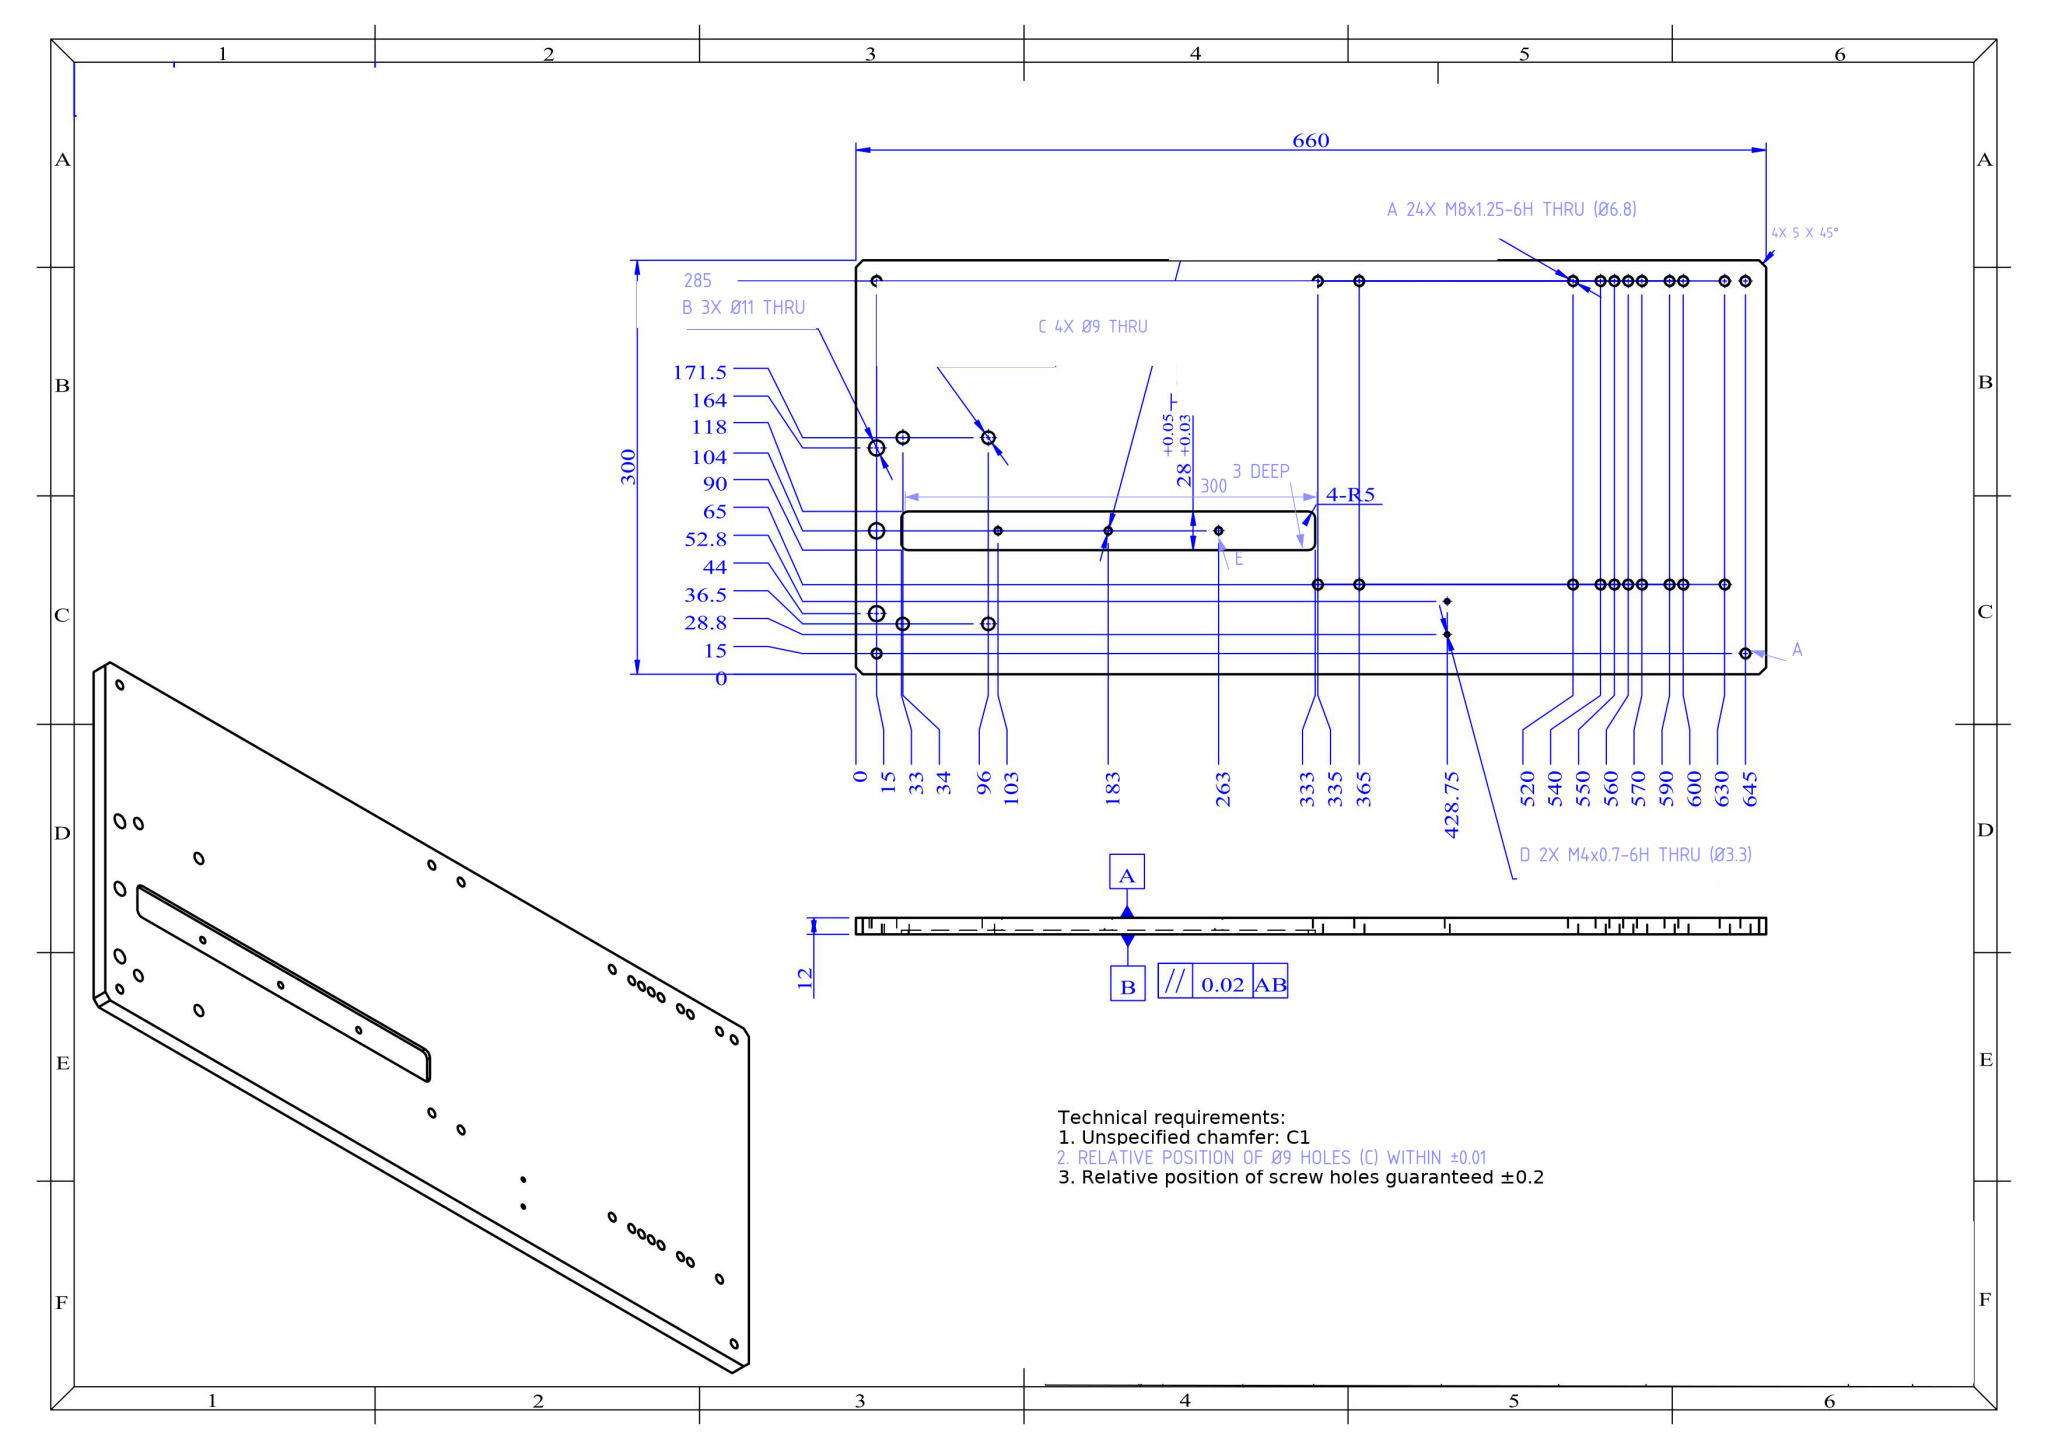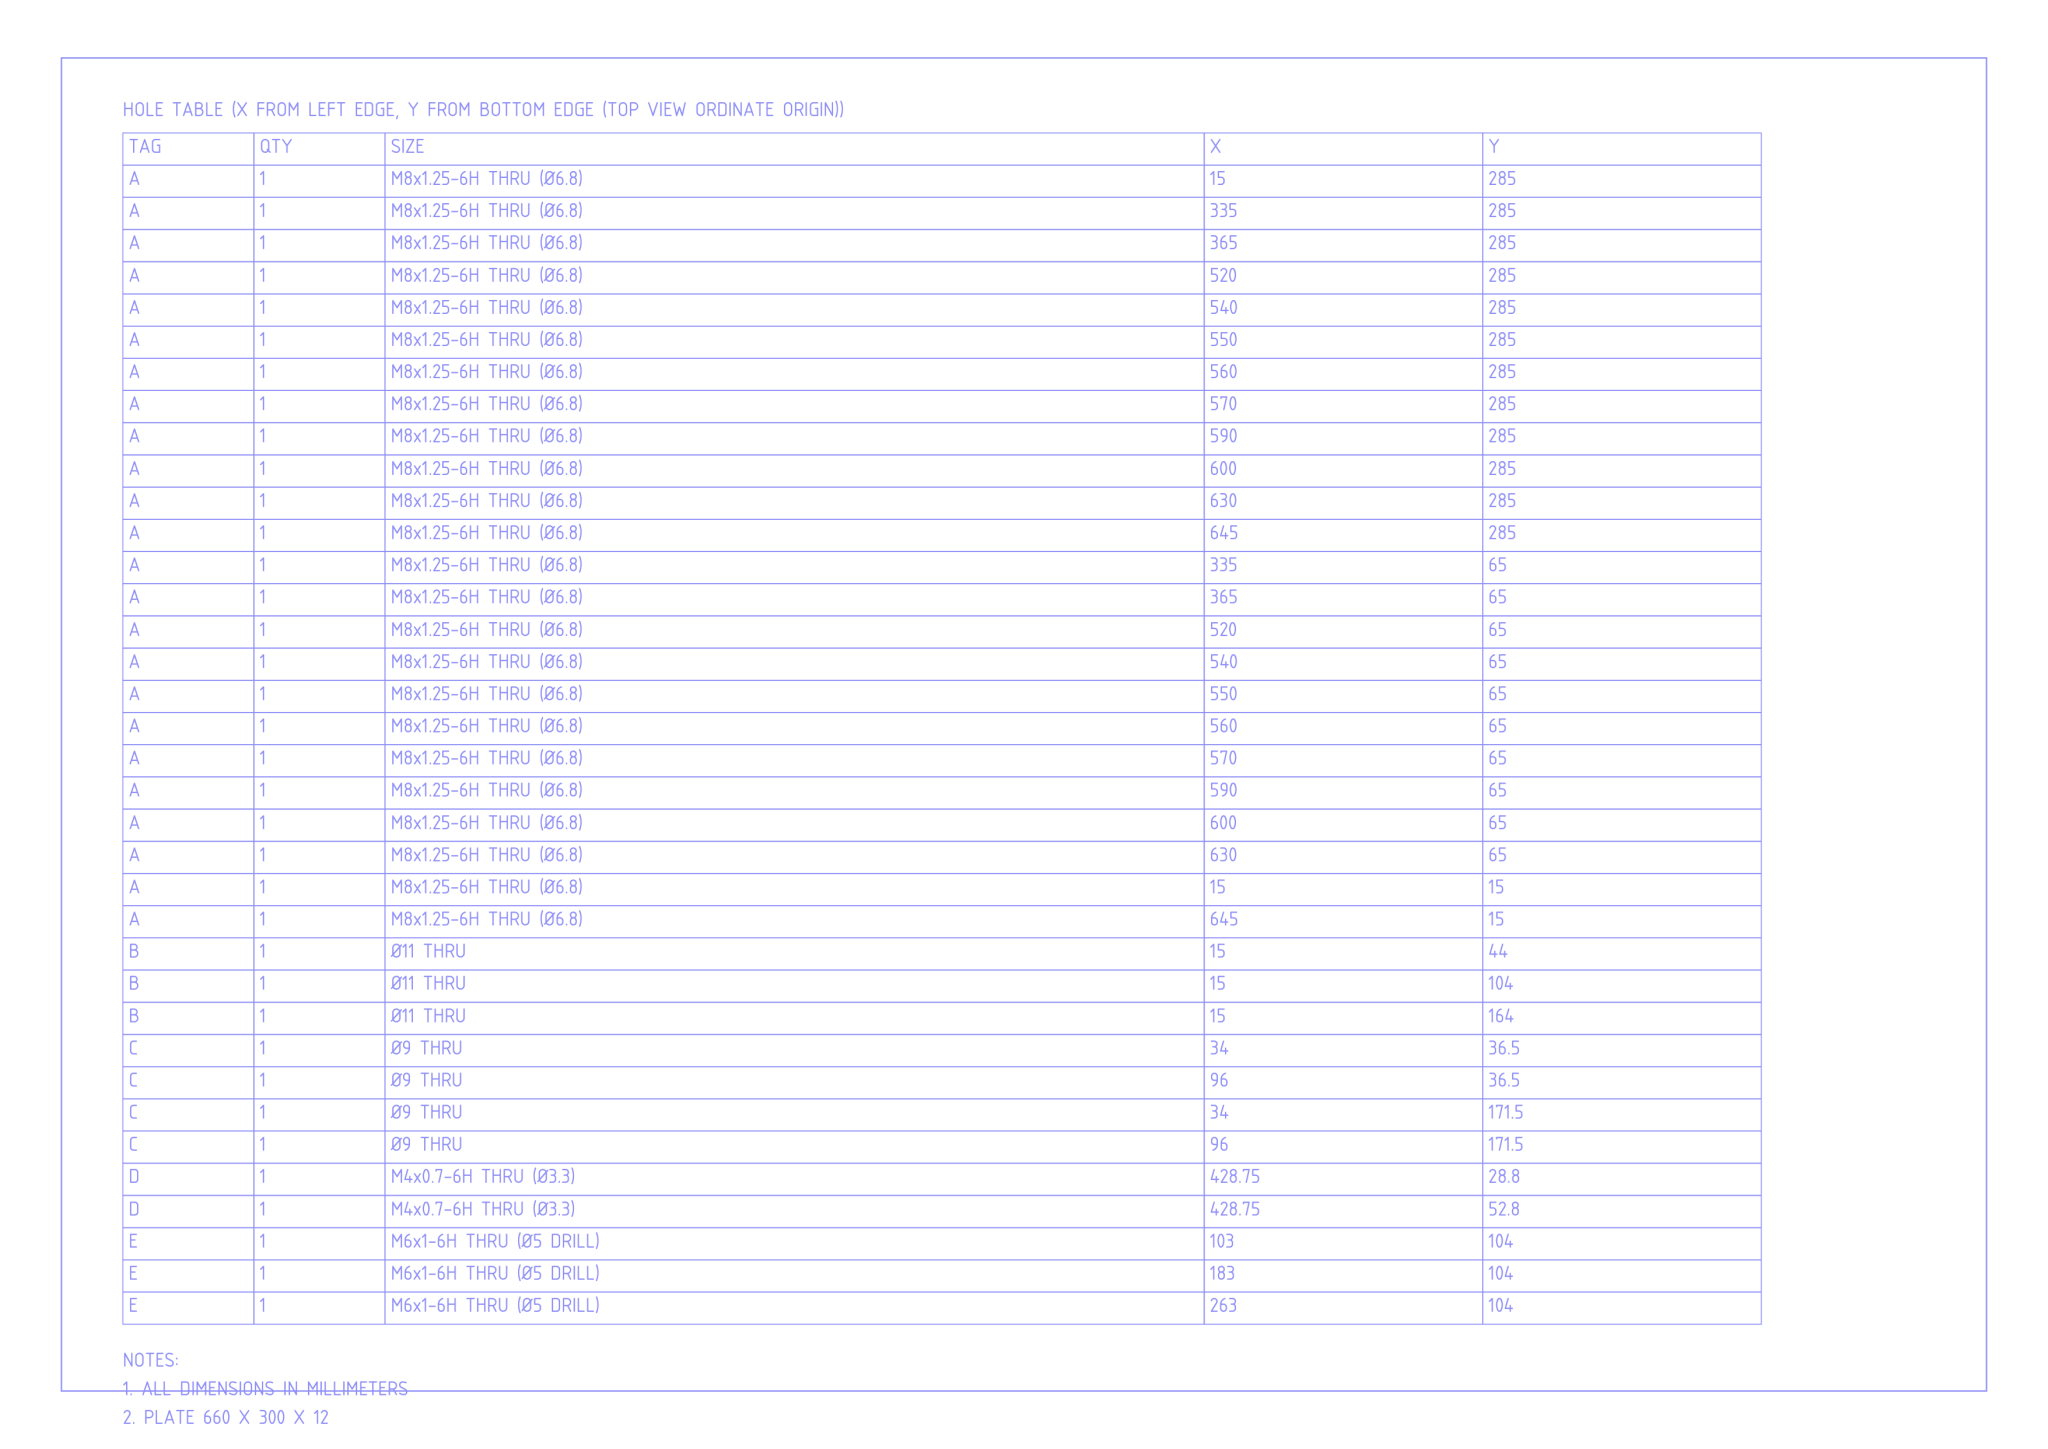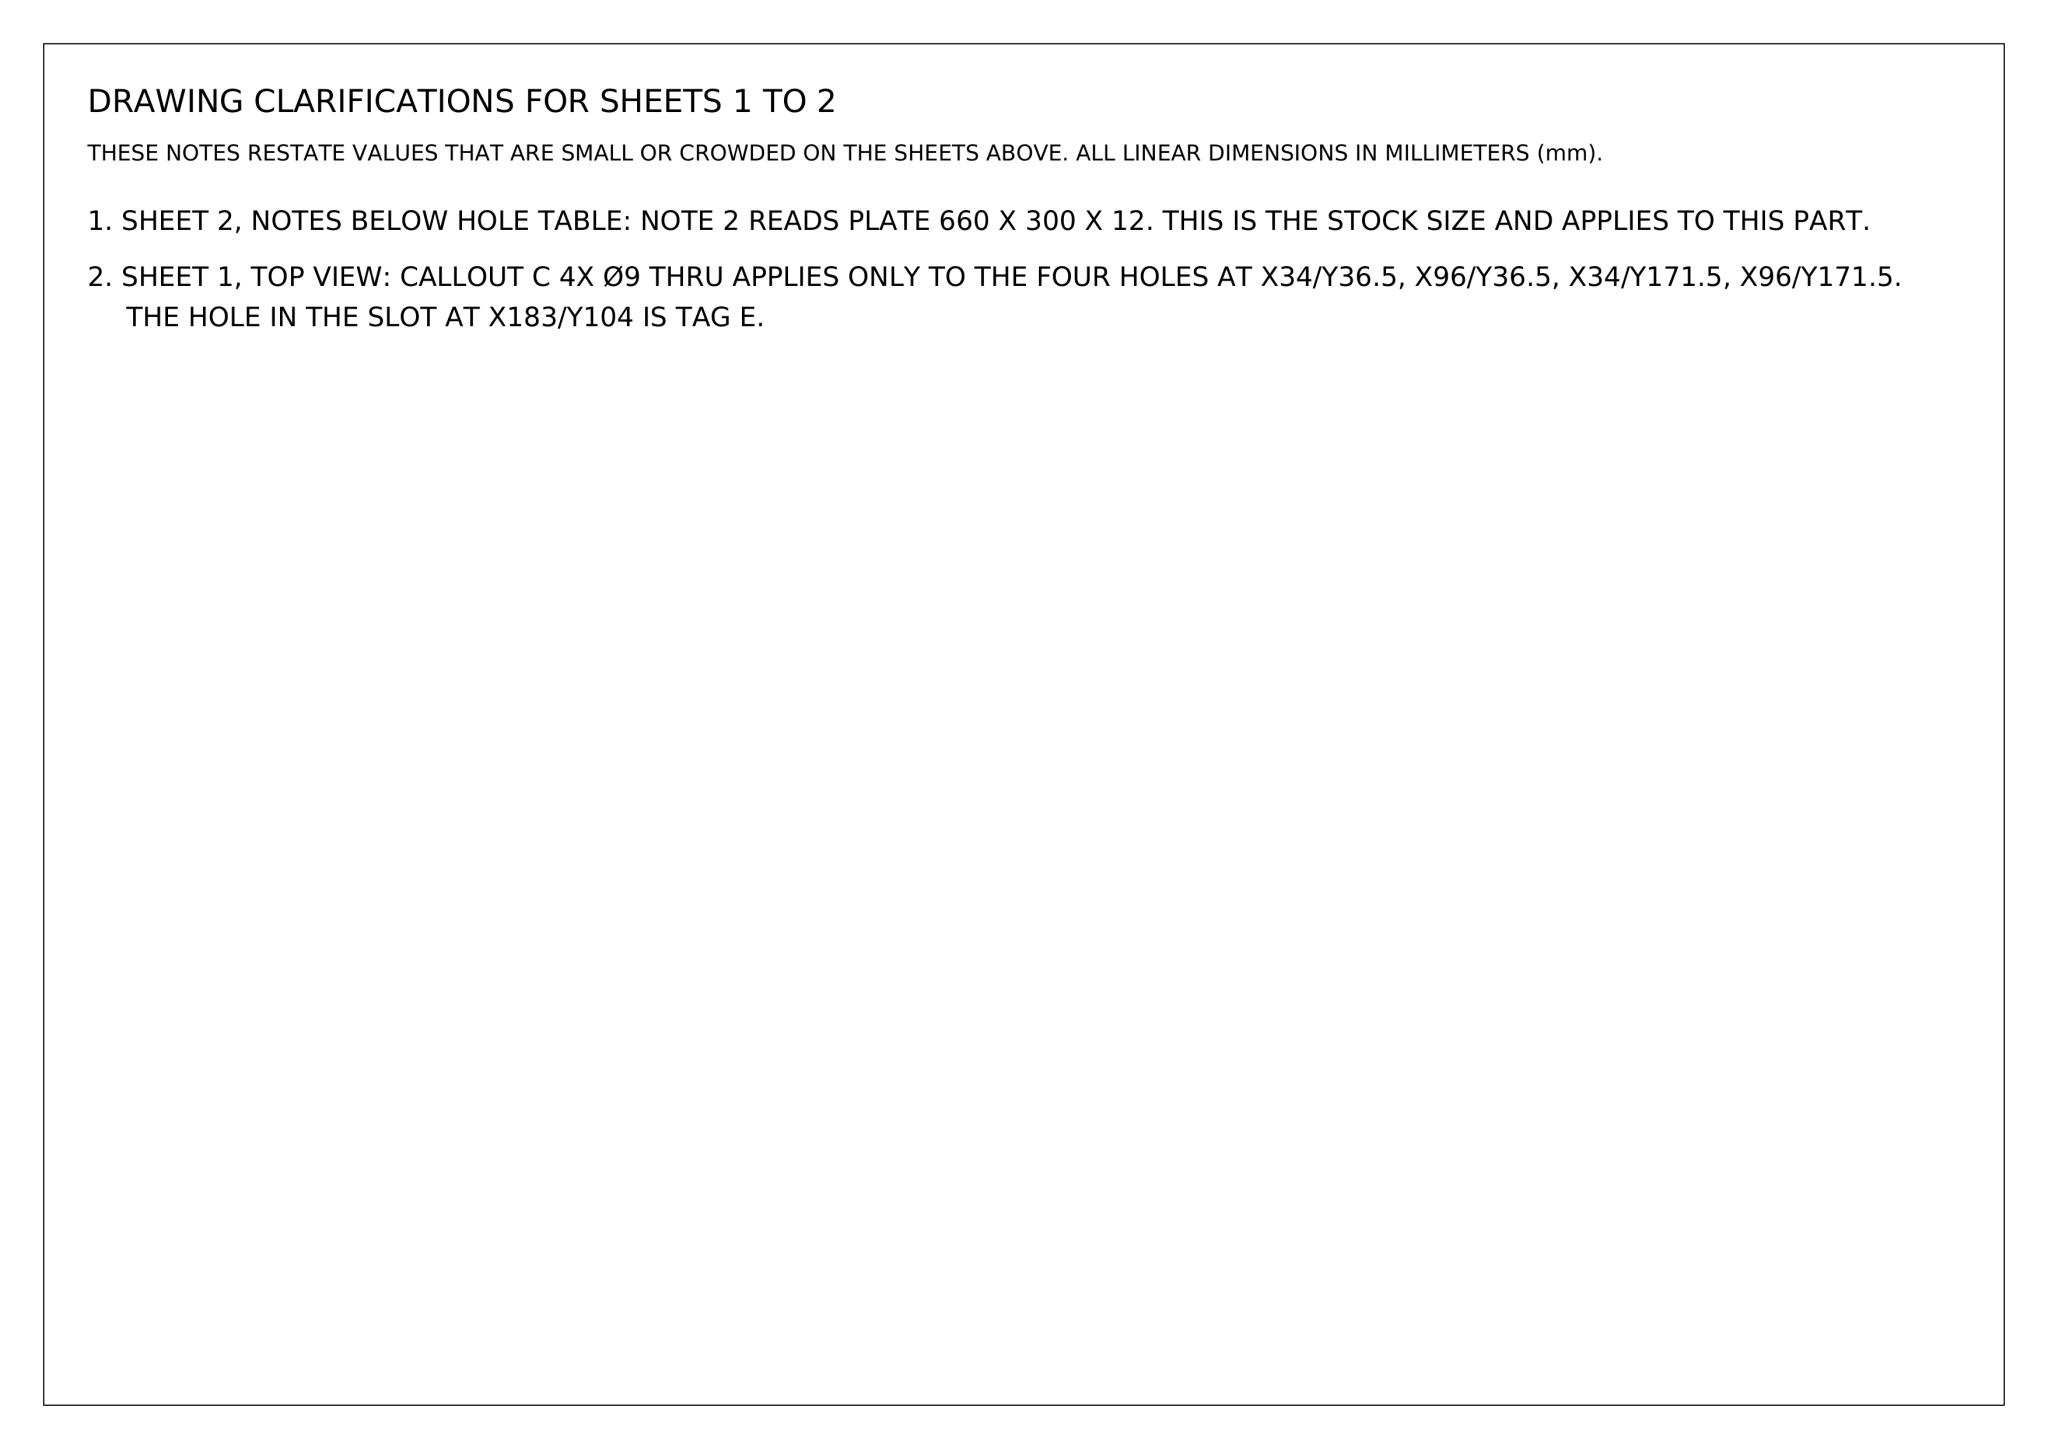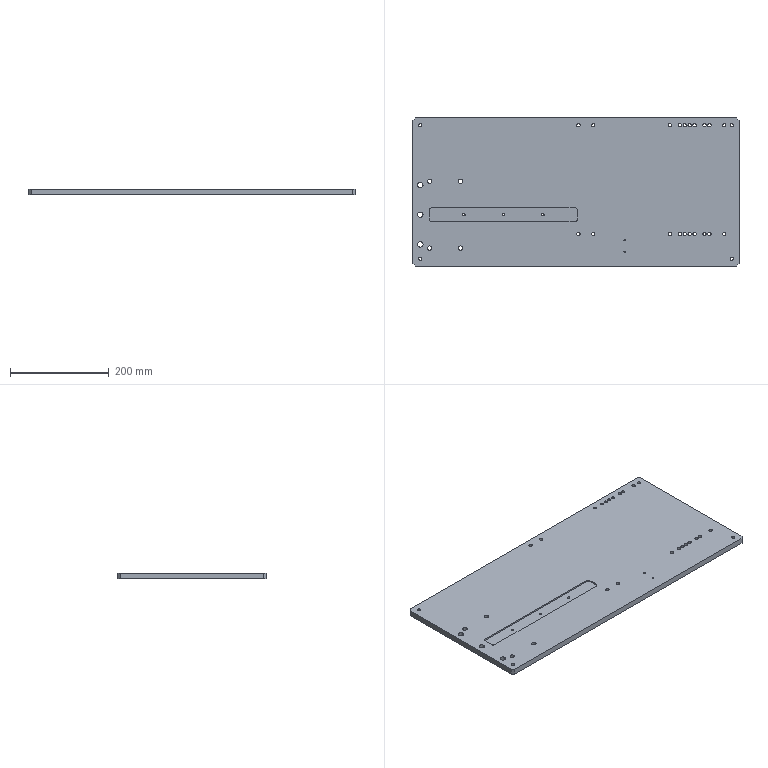Part | NX | mm | 1 solid | 91 faces | box 660 x 300 x 12 mm | volume 2332595 mm3 | cylinder 76 | plane 15 | commonest cylinder face diameters 6.8 x48 9 x8 11 x6 5 x6 3.3 x4 10 x4